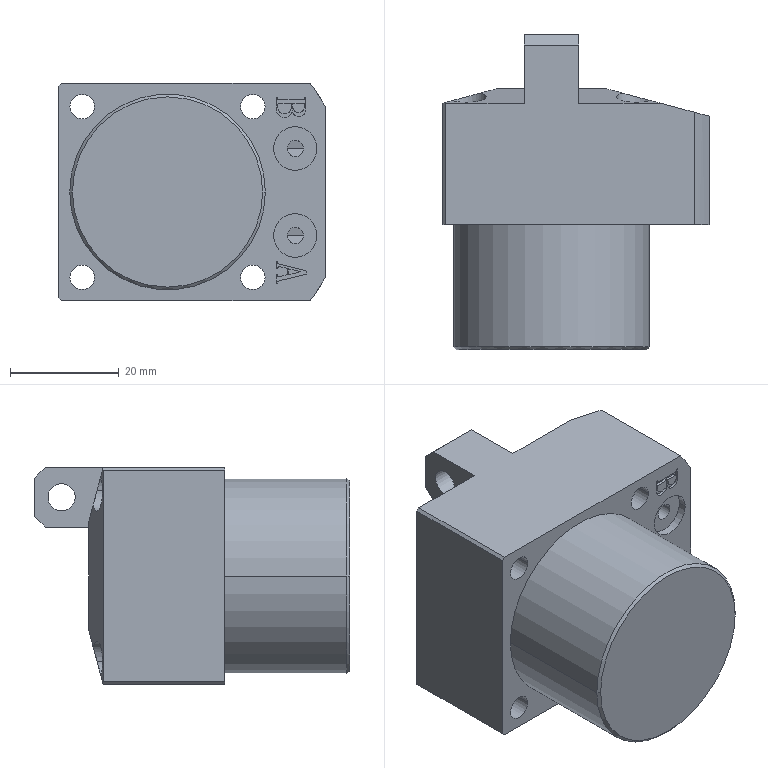Component | SolidWorks | LeverHydraulicRod22-1_HLKA-22GL-1 | 1 solid | 131 faces | volume 55382 mm3 | plane 69 | cylinder 38 | spline 16 | cone 6 | torus 2 | commonest cylinder face diameters 4.5 x8 7.5 x8 7.9 x4 8 x4 3 x4 22 x2 5 x2 10 x2